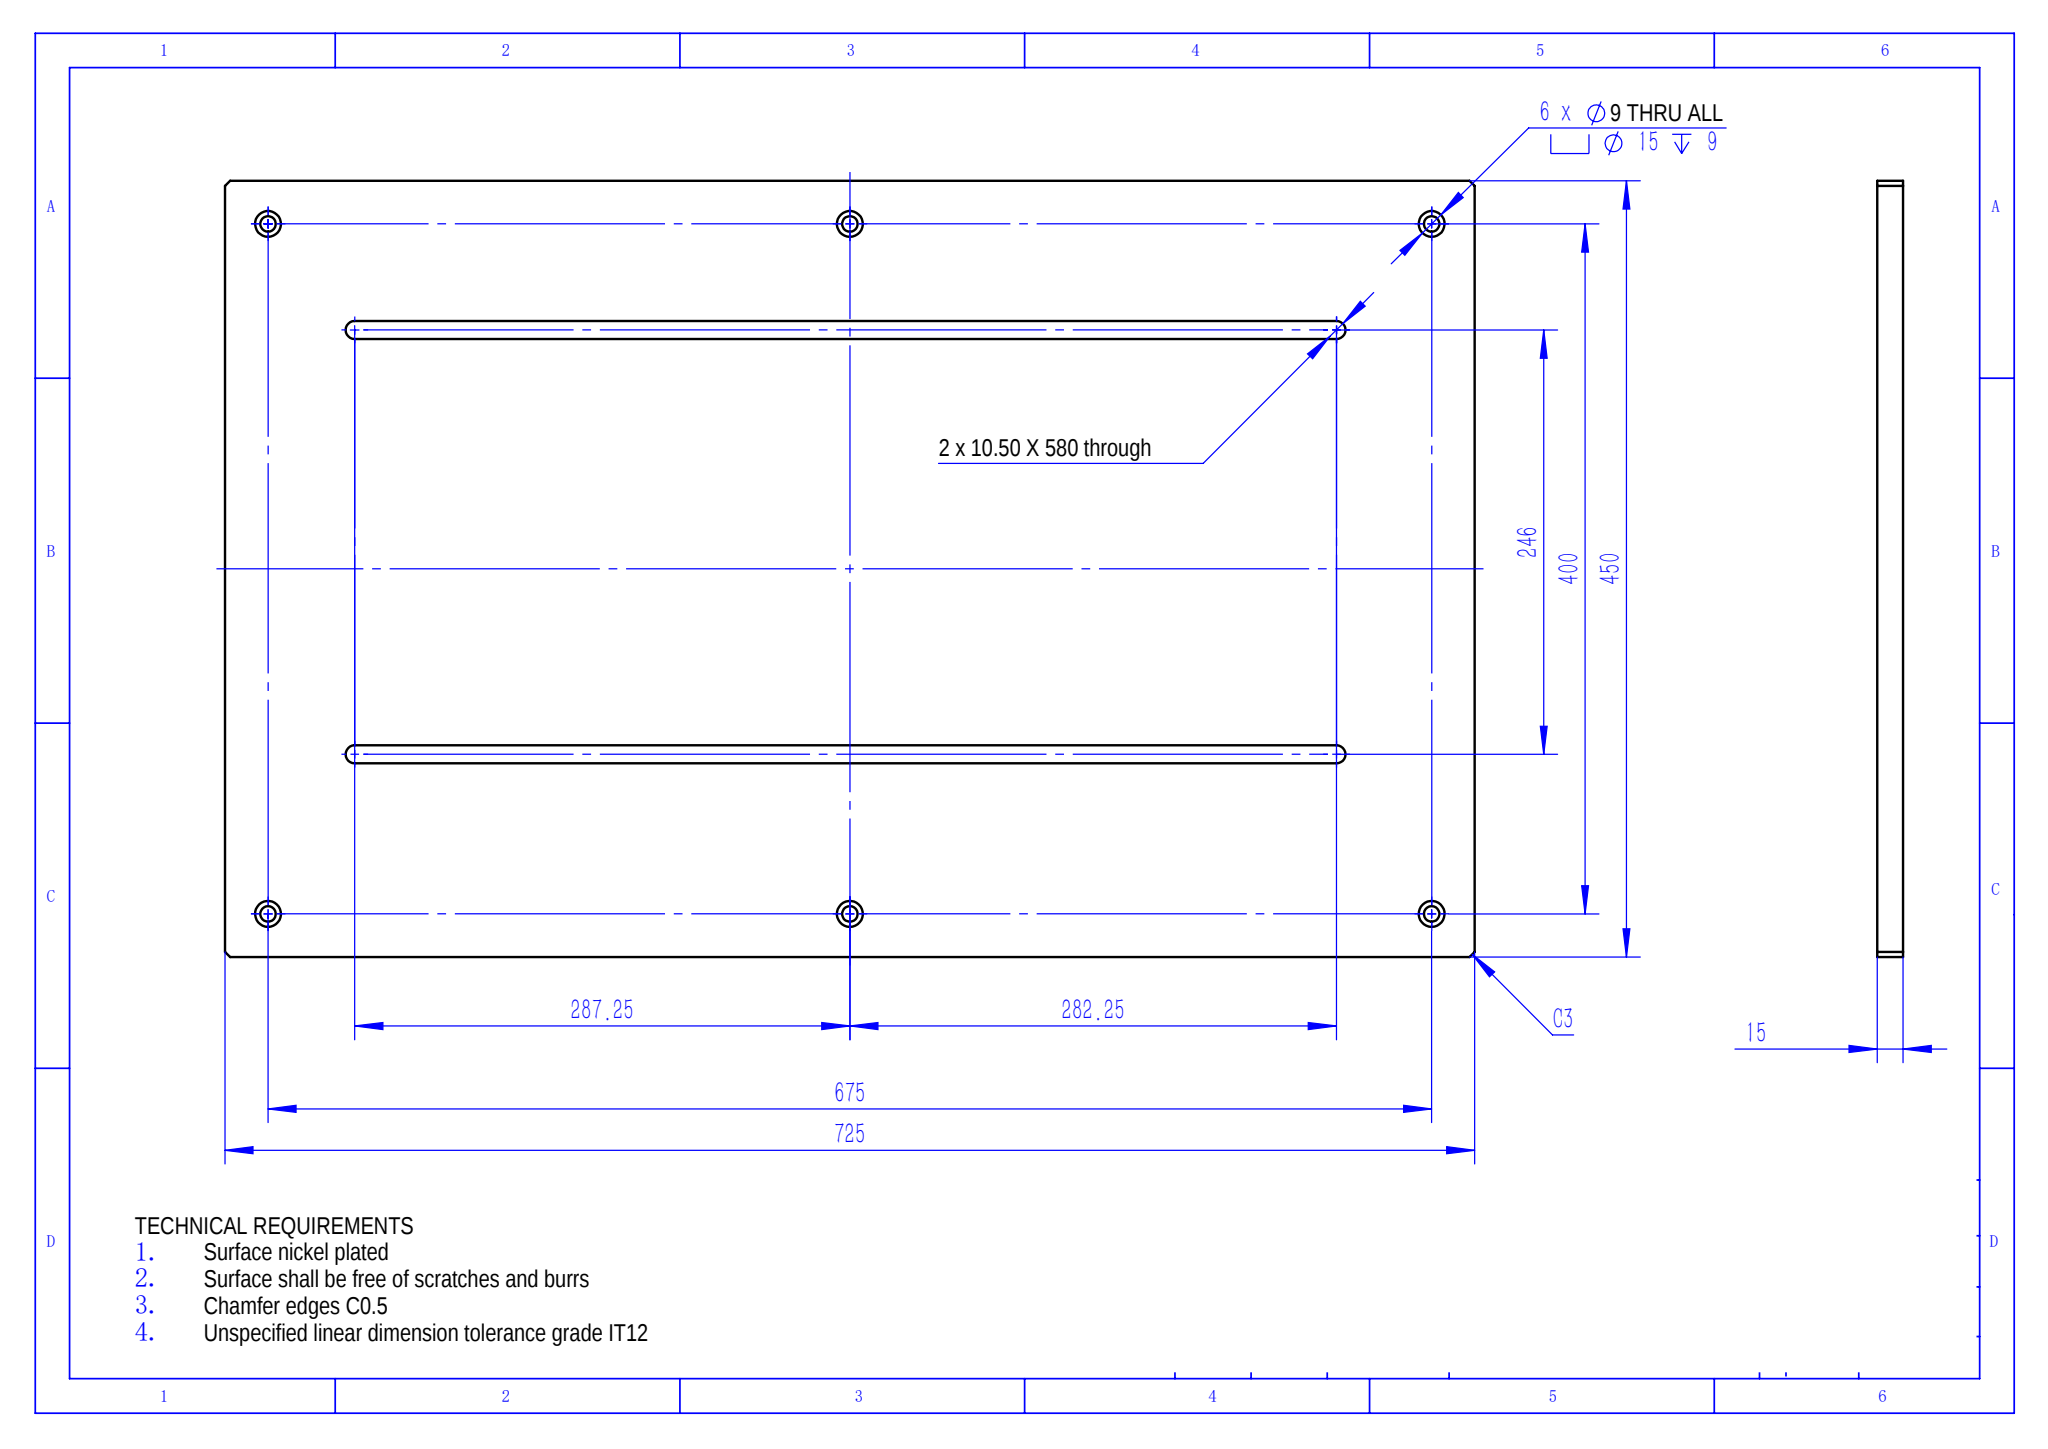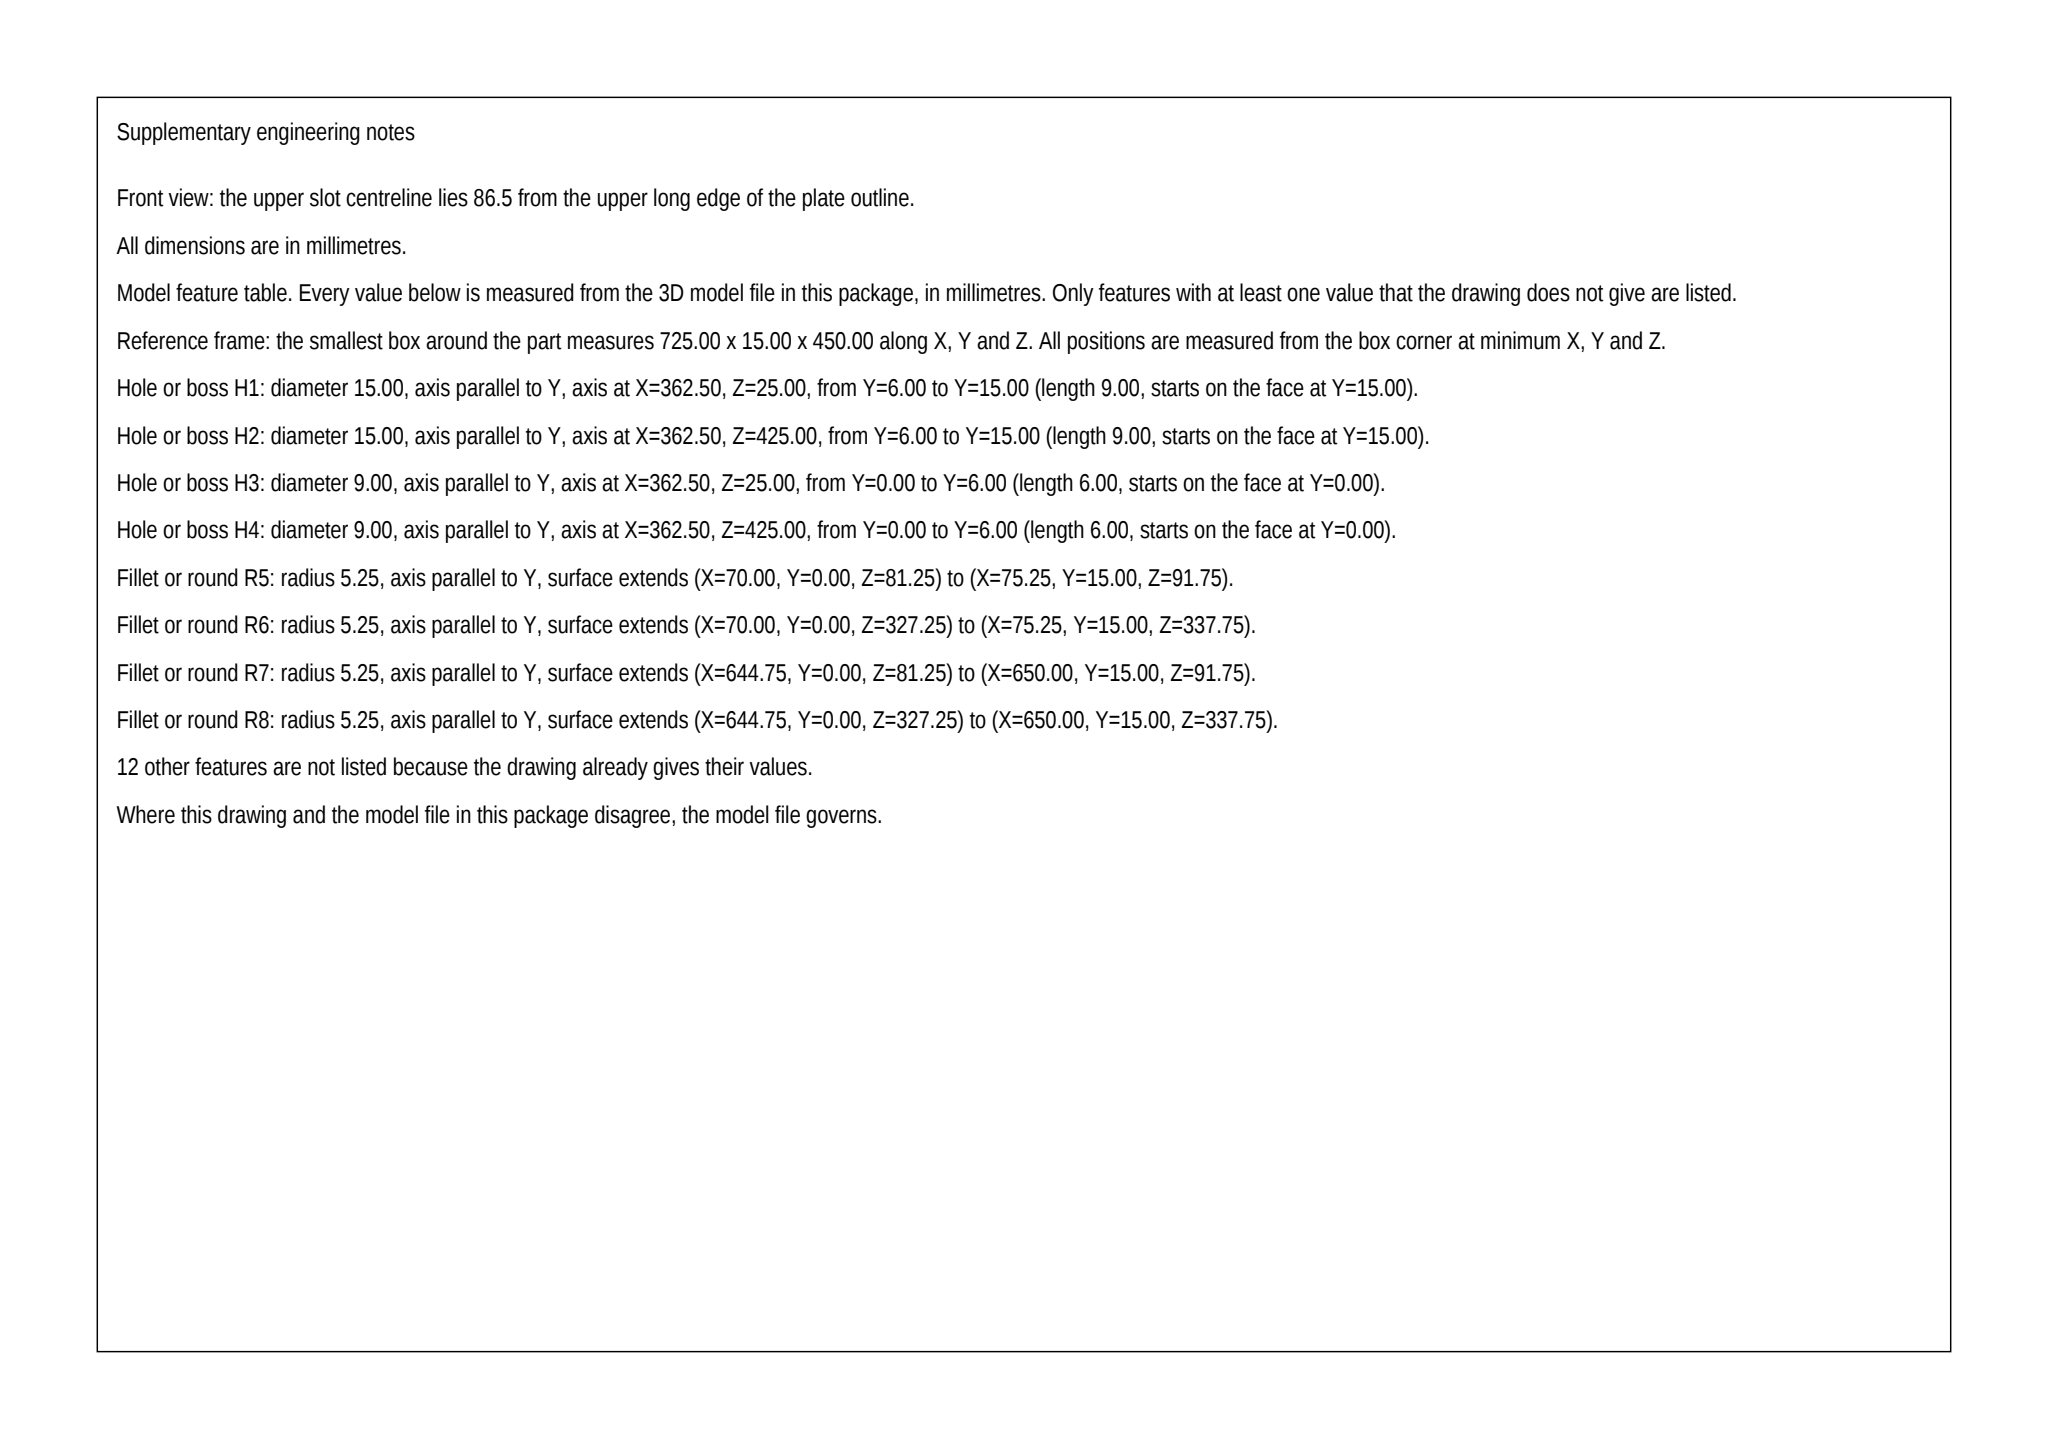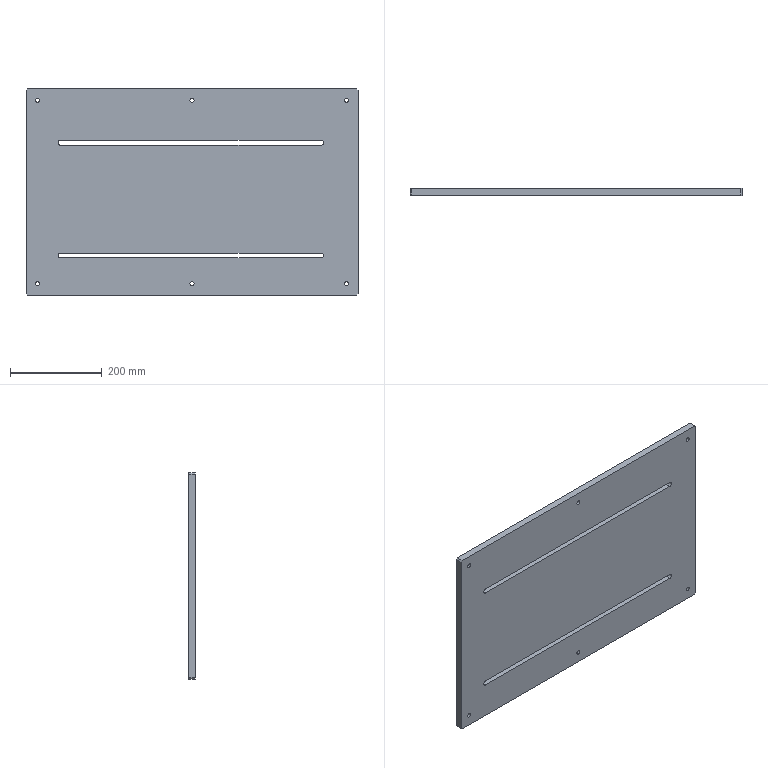Part | SolidWorks | mm | 1 solid | 48 faces | box 725 x 15 x 450 mm | volume 4699657 mm3 | cylinder 28 | plane 20 | commonest cylinder face diameters 15 x12 9 x12 10.5 x4